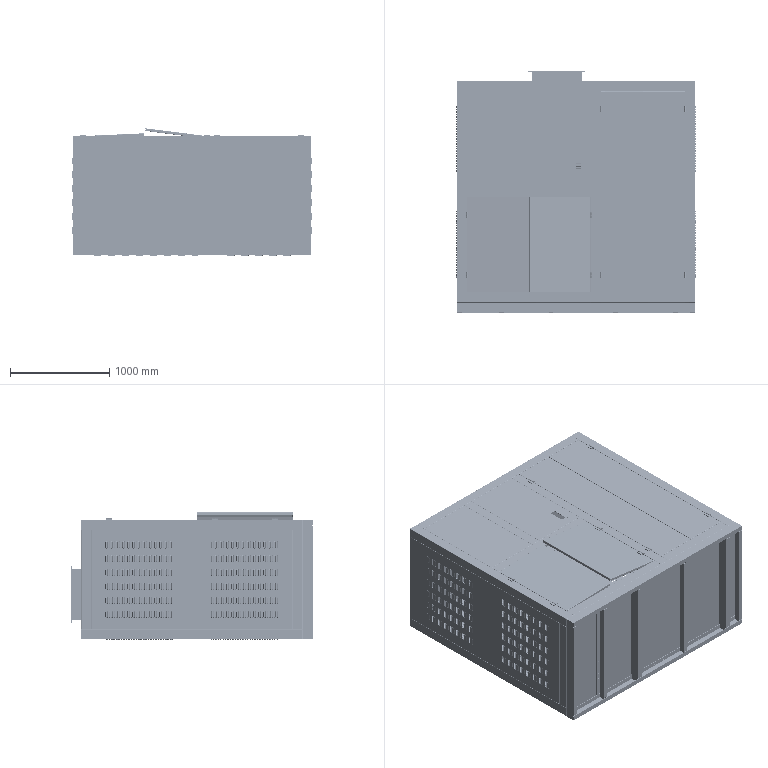Assembly | SolidWorks | mm | 72 component files | 72 solids | 24207 faces | box 2410 x 2430 x 1283.11 mm | volume 69516636 mm3 | plane 10005 | torus 8000 | cylinder 5962 | spline 224 | sphere 16 | commonest cylinder face diameters 10 x3164 14 x2000 2 x288 6 x240 8 x132 12 x64 16 x64 7.5 x4
Bill of materials:
01FrontBase | 1 |  | Long, straight, thin-walled U-channel shown with the open side facing down. It has a flat web and two short side flanges, and no visible holes.
02RearBase | 1 |  | Long, straight, thin-walled U-channel shown with the open side facing up. Small holes are spaced along the flanges, near their top edges.
03LeftSideBase | 1 |  | Straight C-channel standing vertically, opening to the right. The web and flanges appear to end at staggered (offset) heights. One flange has a row of about five small holes.
04RightSideBase | 1 |  | Straight vertical C-channel opening to the left, which appears to be a mirror of the right-opening channels. It has staggered end edges and no visible holes.
05TransformerBaseI | 1 |  | Straight vertical C-channel opening to the right, similar to unnamed part. Its flange holes are in a different pattern: one near the top and three grouped lower down.
06TransformerBaseII | 1 |  | Straight vertical C-channel opening to the left, with staggered ends and no visible holes. It looks the same as unnamed part.
07ResistorBaseI | 1 |  | Straight vertical C-channel opening to the right, similar to the other right-opening channels. It has about four small holes along one flange, spaced fairly evenly in pairs.
08ResistorBaseII | 1 |  | Straight vertical C-channel opening to the left, with staggered ends and no visible holes. It looks the same as unnamed part and unnamed part.
09LeftFrontColumn | 1 |  | Long, straight profile with a stepped, folded cross-section. The end view shows an L-shaped plate with three large round holes, plus thin bent-flange outlines in a Z-like form. Many small holes run along the length, and there are holes near the ends.
10RightFrontColumn | 1 |  | Long, straight profile that appears to be a mirror of unnamed part. The end view shows an L-shaped face with three large holes and Z-like flange outlines. It has fewer holes along its length, mainly small pairs near each end, plus holes on the end face.
11LeftRearColumn | 1 |  | Long, open channel-like profile with stepped or offset flanges. At both ends it has short tabs with small holes, and small holes on the end faces. The end view shows an L-shaped face with three large holes.
12RightRearColumn | 1 |  | Long profile similar to unnamed part, apparently mirrored. It has a row of small holes along one flange, a notched or cut-back flange near the ends, and an end face with holes. The end view shows an L-shaped face with three large holes.
13FrontUpperBeam | 1 |  | Long, straight, thin-walled profile with a right-angle (corner) cross-section. Each leg ends in an outward stepped (Z-jog) flange. An L-shaped end plate with a mitred corner and three round holes closes the end.
14RearUpperBeam | 1 |  | Long, straight, thin-walled right-angle profile with joggled outward flanges on both legs. An L-shaped end plate with three round holes closes the end. It looks like a mirrored or rotated version of the similar long corner profile.
15UpperLeftBeam | 1 |  | Vertical, thin-walled post with a right-angle corner cross-section and joggled outward flanges. L-shaped end plates with three holes sit at the top and bottom.
16UpperRightBeam | 1 |  | Vertical, thin-walled corner-section post with joggled outward flanges and L-shaped end plates with three holes. It appears to be a mirror or rotation of the other corner post.
17FrontMiddleColumn | 1 |  | Long, straight hat-section (top-hat) profile: a raised rectangular channel with an outward flange on each side. A closed end face has two round holes.
18RearMiddleColumn | 1 |  | Long, straight hat-section profile shown inverted, with the channel opening upward and outward flanges at the top. A closed end face has two round holes.
19MiddleUpperBeam | 1 |  | Vertical hat-section post with outward flanges on both sides. End faces at the top and bottom each have two round holes.
20LeftMiddleBeam | 2 |  | Vertical hat-section post: a central channel with an offset flange on each side. End faces at the top and bottom each have two holes.
22BaseLeftSidePlate | 1 |  | Vertical, thin-walled member with a rectangular channel body and a single joggled flange on one side (Z-like, one-sided step). The end face has two round holes.
23BaseRightSidePlate | 1 |  | Vertical, thin-walled member with a channel body and one offset flange on the opposite side from the similar part (mirrored Z-like section). The end face has two round holes.
24BaseFrontSidePlateI | 1 |  | Long, straight, thin-walled profile with a rectangular channel body and one stepped (Z-jog) flange along one edge. The end face has two round holes.
25BaseFrontSidePlateII | 1 |  | Straight, thin-walled profile with a rectangular channel body and one stepped flange along one edge. The end face has two round holes. It appears relatively shorter or wider than the similar long profile.
26BaseRearSidePlateI | 1 |  | Long, slender sheet-metal-style channel with a U-shaped cross-section. One side wall ends in an outward-turned horizontal flange, so the profile looks like a stepped or J shape. The ends are closed by end walls that have holes in them.
27BaseRearSidePlateII | 1 |  | Long sheet-metal-style channel with a U-shaped cross-section, one outward horizontal flange along one side wall, and closed end walls with holes. Similar to part-1f641060 but with fewer side holes.
28FrontMiddleBeam | 1 |  | Long hat-section (omega-profile) channel: a raised crown with two vertical walls and an outward horizontal flange at the base of each wall. The ends are closed by end plates with two holes each.
29RearMiddleBeam | 1 |  | Long hat-section channel shown upside down compared with the previous part: a U-shaped trough with outward horizontal flanges at the top edges. Both ends have end walls with two holes each.
30RearMiddleBeamII | 1 |  | Hat-section trough with outward top flanges and end walls at both ends. It is like part-0d367abd but its side walls have holes, and it looks relatively wider in the top view.
31FrontMiddleColumn | 1 |  | Hat-section channel with the crown on top and outward base flanges. The end walls have two holes each, and there are three small holes along each side wall.
32FrontDoorUpperLeftPlate | 1 |  | Flat rectangular panel or shallow tray with short folded edges around the outside. The edge faces have small, evenly spaced holes. The top face is plain.
33FrontDoorUpperRightPlate | 1 |  | Rectangular panel or shallow tray with short edges and small holes in the edge faces, like part-73c243e1. It also has a rectangular cut-out with four small holes around it near one corner of the top face.
34LeftFront | 1 |  | Rectangular panel with a shallow rim. Along one long edge, a stepped (Z-shaped) offset flange sticks out beyond the main outline. There are two pairs of small holes near the opposite long edge.
35RightFrontDoor | 1 |  | Rectangular panel with a thin perimeter rim and no offset flange. There are two pairs of small holes near one long edge, close to its ends.
36ResistorLeftFrontDoor | 1 |  | Long, narrow rectangular panel with a stepped (Z-shaped) offset flange along one long edge. There are two pairs of small holes near the ends of the other long edge.
37ResistorRightFrontDoor | 1 |  | Long, narrow, flat rectangular panel with a thin edge rim and no offset flange. There are two pairs of small holes near one long edge, at the ends.
38SidePlate | 4 |  | Rectangular thin panel with a shallow perimeter return flange and six parallel rows of closely spaced louver-style slots across the face.
39RearCoverI | 2 |  | Near-square shallow tray-like panel with a perimeter flange and five parallel bands of louver-style slots.
40RearCoverII | 2 |  | Rectangular shallow tray-like panel with a perimeter flange and eight parallel bands of louver-style slots.
41TopPlateI | 1 |  | Plain rectangular panel with a shallow perimeter flange and a ring of small holes near the edges; no other openings.
42TopPlateII | 1 |  | Rectangular panel with a shallow perimeter flange, small perimeter holes, and one large square/rectangular through-cutout offset toward one corner.
43BottomPlate | 1 |  | Very thin flat rectangular sheet with no flanges, perforated by small holes arranged in four vertical column groups.
ActuatorGasket | 1 |  | Elongated rectangular cover with bent-down flanges on the edges, a rectangular through-cutout near one end surrounded by four small holes, and one larger round hole in an end flange.
ColumnBlockingPlate | 4 |  | Bent sheet bracket: a large flat plate with a short perpendicular base tab and a perpendicular side tab, each tab carrying one round hole.
DoorHinge1 | 8 |  | Small rectangular block/plate with rounded edges, two hollow cylindrical knuckles along one long edge, and two cylindrical pins projecting from the underside.
DoorHinge2 | 8 |  | Rectangular block/plate with two hollow cylindrical knuckles offset along one long edge and two cylindrical pins on the underside; similar to, but laid out differently from, unnamed part.
DoorHinge3 | 2 |  | Plain solid cylindrical rod with flat ends and no visible features.
Riser | 1 |  | Open rectangular sleeve/frame (four walls, open both ends) with a thin outward perimeter flange at one end.
Mates:
1. coincident | 03LeftSideBase-2 face at (-123.527, -39.54, 1231.607) dir (0, 1, 0) | 01FrontBase-1 face at (2276.473, -39.54, 1237.107) dir (0, 1, 0)
2. coincident | 03LeftSideBase-2 face at (-75.527, -45.04, 1231.607) dir (0, 0, 1) | 01FrontBase-1 face at (2276.473, -139.54, 1231.607) dir (0, 0, -1)
3. coincident | 03LeftSideBase-2 face at (-123.527, -139.54, 1231.607) dir (-1, 0, 0) | 01FrontBase-1 face at (-123.527, -45.04, 1189.107) dir (-1, 0, 0)
4. coincident | 03LeftSideBase-2 face at (-75.527, -45.04, 42.607) dir (0, 0, -1) | 02RearBase-1 face at (-123.527, -139.54, 42.607) dir (0, 0, 1)
5. coincident | 03LeftSideBase-2 face at (-123.527, -39.54, 1231.607) dir (0, 1, 0) | 02RearBase-1 face at (-123.527, -39.54, 37.107) dir (0, 1, 0)
6. coincident | 03LeftSideBase-2 face at (-123.527, -139.54, 1231.607) dir (-1, 0, 0) | 02RearBase-1 face at (-123.527, -45.04, 85.107) dir (-1, 0, 0)
7. coincident | 01FrontBase-1 face at (2276.473, -45.04, 1189.107) dir (1, 0, 0) | 04RightSideBase-3 face at (2276.473, -139.54, 42.607) dir (1, 0, 0)
8. coincident | 01FrontBase-1 face at (2276.473, -39.54, 1237.107) dir (0, 1, 0) | 04RightSideBase-3 face at (2276.473, -39.54, 42.607) dir (0, 1, 0)
9. coincident | 02RearBase-1 face at (-123.527, -139.54, 42.607) dir (0, 0, 1) | 04RightSideBase-3 face at (2228.473, -45.04, 42.607) dir (0, 0, -1)
10. coincident | 02RearBase-1 face at (-123.527, -39.54, 37.107) dir (0, 1, 0) | 05TransformerBaseI-1 face at (801.473, -39.54, 1231.607) dir (0, 1, 0)
11. coincident | 02RearBase-1 face at (-123.527, -139.54, 42.607) dir (0, 0, 1) | 05TransformerBaseI-1 face at (849.473, -45.04, 42.607) dir (0, 0, -1)
12. coincident | 02RearBase-1 face at (-123.527, -39.54, 37.107) dir (0, 1, 0) | 06TransformerBaseII-1 face at (351.473, -39.54, 42.607) dir (0, 1, 0)
13. coincident | 01FrontBase-1 face at (2276.473, -139.54, 1231.607) dir (0, 0, -1) | 06TransformerBaseII-1 face at (303.473, -45.04, 1231.607) dir (0, 0, 1)
14. coincident | 02RearBase-1 face at (-123.527, -39.54, 37.107) dir (0, 1, 0) | 07ResistorBaseI-1 face at (2053.973, -39.54, 1231.607) dir (0, 1, 0)
15. coincident | 01FrontBase-1 face at (2276.473, -139.54, 1231.607) dir (0, 0, -1) | 07ResistorBaseI-1 face at (2101.973, -45.04, 1231.607) dir (0, 0, 1)
16. coincident | 01FrontBase-1 face at (2276.473, -39.54, 1237.107) dir (0, 1, 0) | 09LeftFrontColumn-2 face at (-95.527, -39.54, 1140.107) dir (0, -1, 0)
17. coincident | 01FrontBase-1 face at (2276.473, -139.54, 1237.107) dir (0, 0, 1) | 09LeftFrontColumn-2 face at (-25.527, 2190.46, 1237.107) dir (0, 0, 1)
18. coincident | 03LeftSideBase-2 face at (-123.527, -139.54, 1231.607) dir (-1, 0, 0) | 09LeftFrontColumn-2 face at (-123.527, 2190.46, 1235.107) dir (-1, 0, 0)
19. coincident | 09LeftFrontColumn-2 face at (-123.527, 2190.46, 1235.107) dir (0, 1, 0) | ColumnBlockingPlate-1 face at (-23.527, 2190.46, 1235.107) dir (0, 1, 0)
20. coincident | 09LeftFrontColumn-2 face at (-121.527, 2190.46, 1235.107) dir (1, 0, 0) | ColumnBlockingPlate-1 face at (-121.527, 2188.46, 1137.107) dir (-1, 0, 0)
21. coincident | 09LeftFrontColumn-2 face at (-25.527, 2190.46, 1235.107) dir (0, 0, -1) | ColumnBlockingPlate-1 face at (-23.527, 2188.46, 1235.107) dir (0, 0, 1)
22. coincident | 04RightSideBase-3 face at (2276.473, -139.54, 42.607) dir (1, 0, 0) | 10RightFrontColumn-1 face at (2276.473, 2190.46, 1139.107) dir (1, 0, 0)
23. coincident | 01FrontBase-1 face at (2276.473, -139.54, 1237.107) dir (0, 0, 1) | 10RightFrontColumn-1 face at (2274.473, 2190.46, 1237.107) dir (0, 0, 1)
24. coincident | 01FrontBase-1 face at (2276.473, -39.54, 1237.107) dir (0, 1, 0) | 10RightFrontColumn-1 face at (2179.473, -39.54, 1209.107) dir (0, -1, 0)
25. coincident | 10RightFrontColumn-1 face at (2274.473, 2190.46, 1235.107) dir (0, 0, -1) | ColumnBlockingPlate-2 face at (2176.473, 2188.46, 1235.107) dir (0, 0, 1)
26. coincident | 10RightFrontColumn-1 face at (2274.473, 2190.46, 1139.107) dir (-1, 0, 0) | ColumnBlockingPlate-2 face at (2274.473, 2188.46, 1137.107) dir (1, 0, 0)
27. coincident | 10RightFrontColumn-1 face at (2273.473, 2190.46, 1234.107) dir (0, 1, 0) | ColumnBlockingPlate-2 face at (2274.473, 2190.46, 1137.107) dir (0, 1, 0)
28. coincident | 03LeftSideBase-2 face at (-123.527, -139.54, 1231.607) dir (-1, 0, 0) | 11LeftRearColumn-1 face at (-123.527, 2190.46, 135.107) dir (-1, 0, 0)
29. coincident | 02RearBase-1 face at (-123.527, -139.54, 37.107) dir (0, 0, -1) | 11LeftRearColumn-1 face at (-121.527, 2190.46, 37.107) dir (0, 0, -1)
30. coincident | 03LeftSideBase-2 face at (-123.527, -39.54, 1231.607) dir (0, 1, 0) | 11LeftRearColumn-1 face at (-26.527, -39.54, 65.107) dir (0, -1, 0)
31. coincident | 11LeftRearColumn-1 face at (-23.527, 2190.46, 39.107) dir (0, 1, 0) | ColumnBlockingPlate-3 face at (-121.527, 2190.46, 137.107) dir (0, 1, 0)
32. coincident | 11LeftRearColumn-1 face at (-121.527, 2190.46, 135.107) dir (1, 0, 0) | ColumnBlockingPlate-3 face at (-121.527, 2188.46, 137.107) dir (-1, 0, 0)
33. coincident | 11LeftRearColumn-1 face at (-121.527, 2190.46, 39.107) dir (0, 0, 1) | ColumnBlockingPlate-3 face at (-23.527, 2188.46, 39.107) dir (0, 0, -1)
34. coincident | 04RightSideBase-3 face at (2276.473, -139.54, 42.607) dir (1, 0, 0) | 12RightRearColumn-2 face at (2276.473, 2190.46, 39.107) dir (1, 0, 0)
35. coincident | 02RearBase-1 face at (-123.527, -139.54, 37.107) dir (0, 0, -1) | 12RightRearColumn-2 face at (2178.473, 2190.46, 37.107) dir (0, 0, -1)
36. coincident | 04RightSideBase-3 face at (2276.473, -39.54, 42.607) dir (0, 1, 0) | 12RightRearColumn-2 face at (2248.473, -39.54, 134.107) dir (0, -1, 0)
37. coincident | 12RightRearColumn-2 face at (2276.473, 2190.46, 39.107) dir (0, 1, 0) | ColumnBlockingPlate-4 face at (2176.473, 2190.46, 39.107) dir (0, 1, 0)
38. coincident | 12RightRearColumn-2 face at (2178.473, 2190.46, 39.107) dir (0, 0, 1) | ColumnBlockingPlate-4 face at (2176.473, 2188.46, 39.107) dir (0, 0, -1)
39. coincident | 12RightRearColumn-2 face at (2274.473, 2190.46, 39.107) dir (-1, 0, 0) | ColumnBlockingPlate-4 face at (2274.473, 2188.46, 137.107) dir (1, 0, 0)
40. coincident | 09LeftFrontColumn-2 face at (-25.527, 2190.46, 1237.107) dir (0, 0, 1) | 13FrontUpperBeam-1 face at (2176.473, 2092.46, 1237.107) dir (0, 0, 1)
41. coincident | ColumnBlockingPlate-1 face at (-23.527, 2190.46, 1235.107) dir (0, 1, 0) | 13FrontUpperBeam-1 face at (2176.473, 2190.46, 1235.107) dir (0, 1, 0)
42. coincident | 10RightFrontColumn-1 face at (2176.473, 2190.46, 1235.107) dir (-1, 0, 0) | 13FrontUpperBeam-1 face at (2176.473, 2187.46, 1209.107) dir (1, 0, 0)
43. coincident | ColumnBlockingPlate-4 face at (2176.473, 2190.46, 39.107) dir (0, 1, 0) | 14RearUpperBeam-1 face at (2176.473, 2190.46, 135.107) dir (0, 1, 0)
44. coincident | 12RightRearColumn-2 face at (2178.473, 2190.46, 37.107) dir (0, 0, -1) | 14RearUpperBeam-1 face at (2176.473, 2188.46, 37.107) dir (0, 0, -1)
45. coincident | 12RightRearColumn-2 face at (2176.473, -39.54, 67.107) dir (-1, 0, 0) | 14RearUpperBeam-1 face at (2176.473, 2093.46, 65.107) dir (1, 0, 0)
46. coincident | ColumnBlockingPlate-1 face at (-23.527, 2190.46, 1235.107) dir (0, 1, 0) | 15UpperLeftBeam-1 face at (-25.527, 2190.46, 137.107) dir (0, 1, 0)
47. coincident | 09LeftFrontColumn-2 face at (-121.527, 2190.46, 1137.107) dir (0, 0, -1) | 15UpperLeftBeam-1 face at (-95.527, 2093.46, 1137.107) dir (0, 0, 1)
48. coincident | 11LeftRearColumn-1 face at (-93.527, -39.54, 137.107) dir (0, 0, 1) | 15UpperLeftBeam-1 face at (-95.527, 2093.46, 137.107) dir (0, 0, -1)
49. coincident | 11LeftRearColumn-1 face at (-123.527, 2190.46, 135.107) dir (-1, 0, 0) | 15UpperLeftBeam-1 face at (-123.527, 2188.46, 137.107) dir (-1, 0, 0)
50. coincident | 02RearBase-1 face at (-123.527, -39.54, 37.107) dir (0, 1, 0) | 18RearMiddleColumn-2 face at (1323.473, -39.54, 39.107) dir (0, -1, 0)
51. coincident | 02RearBase-1 face at (-123.527, -139.54, 37.107) dir (0, 0, -1) | 18RearMiddleColumn-2 face at (1324.473, -39.54, 37.107) dir (0, 0, -1)
52. distance | 18RearMiddleColumn-2 face at (1326.473, 2090.46, 67.107) dir (1, 0, 0) | 12RightRearColumn-2 face at (2276.473, 2190.46, 39.107) dir (1, 0, 0)
53. coincident | 01FrontBase-1 face at (2276.473, -39.54, 1237.107) dir (0, 1, 0) | 17FrontMiddleColumn-2 face at (1229.473, -39.54, 1235.107) dir (0, -1, 0)
54. coincident | 01FrontBase-1 face at (2276.473, -139.54, 1237.107) dir (0, 0, 1) | 17FrontMiddleColumn-2 face at (1228.473, -39.54, 1237.107) dir (0, 0, 1)
55. distance | 17FrontMiddleColumn-2 face at (1326.473, -39.54, 1235.107) dir (1, 0, 0) | 10RightFrontColumn-1 face at (2276.473, 2190.46, 1139.107) dir (1, 0, 0)
56. coincident | 14RearUpperBeam-1 face at (2176.473, 2190.46, 135.107) dir (0, 1, 0) | 16UpperRightBeam-1 face at (2178.473, 2190.46, 1137.107) dir (0, 1, 0)
57. coincident | 12RightRearColumn-2 face at (2276.473, 2190.46, 39.107) dir (1, 0, 0) | 16UpperRightBeam-1 face at (2276.473, 2188.46, 1137.107) dir (1, 0, 0)
58. coincident | 12RightRearColumn-2 face at (2274.473, 2190.46, 137.107) dir (0, 0, 1) | 16UpperRightBeam-1 face at (2248.473, 2093.46, 137.107) dir (0, 0, -1)
59. coincident | 14RearUpperBeam-1 face at (-23.527, 2160.46, 137.107) dir (0, 0, 1) | 19MiddleUpperBeam-1 face at (1323.473, 2188.46, 137.107) dir (0, 0, -1)
60. coincident | 13FrontUpperBeam-1 face at (2176.473, 2190.46, 1235.107) dir (0, 1, 0) | 19MiddleUpperBeam-1 face at (1228.473, 2190.46, 1137.107) dir (0, 1, 0)
61. distance | 19MiddleUpperBeam-1 face at (1226.473, 2160.46, 137.107) dir (-1, 0, 0) | 15UpperLeftBeam-1 face at (-23.527, 2160.46, 1137.107) dir (1, 0, 0)
62. coincident | 11LeftRearColumn-1 face at (-93.527, -39.54, 137.107) dir (0, 0, 1) | 20LeftMiddleBeam-1 face at (-121.527, 1122.46, 137.107) dir (0, 0, -1)
63. coincident | 11LeftRearColumn-1 face at (-123.527, 2190.46, 135.107) dir (-1, 0, 0) | 20LeftMiddleBeam-1 face at (-123.527, 1027.46, 1137.107) dir (-1, 0, 0)
64. distance | 03LeftSideBase-2 face at (-123.527, -39.54, 1231.607) dir (0, 1, 0) | 20LeftMiddleBeam-1 face at (-93.527, 1025.46, 137.107) dir (0, -1, 0)
65. coincident | 12RightRearColumn-2 face at (2276.473, 2190.46, 39.107) dir (1, 0, 0) | 20LeftMiddleBeam-2 face at (2276.473, 1027.46, 137.107) dir (1, 0, 0)
66. coincident | 10RightFrontColumn-1 face at (2246.473, -39.54, 1137.107) dir (0, 0, -1) | 20LeftMiddleBeam-2 face at (2274.473, 1122.46, 1137.107) dir (0, 0, 1)
67. distance | 04RightSideBase-3 face at (2276.473, -39.54, 42.607) dir (0, 1, 0) | 20LeftMiddleBeam-2 face at (2246.473, 1025.46, 1137.107) dir (0, -1, 0)
68. coincident | 09LeftFrontColumn-2 face at (-121.527, 2190.46, 1137.107) dir (0, 0, -1) | 22BaseLeftSidePlate-1 face at (-91.527, -5039.54, 1137.107) dir (0, 0, 1)
69. coincident | 03LeftSideBase-2 face at (-123.527, -39.54, 1231.607) dir (0, 1, 0) | 22BaseLeftSidePlate-1 face at (-91.527, -39.54, -4862.893) dir (0, -1, 0)
70. coincident | 03LeftSideBase-2 face at (-123.527, -139.54, 1231.607) dir (-1, 0, 0) | 22BaseLeftSidePlate-1 face at (-123.527, 60.46, 1137.107) dir (-1, 0, 0)
71. coincident | 04RightSideBase-3 face at (2276.473, -139.54, 42.607) dir (1, 0, 0) | 23BaseRightSidePlate-1 face at (2276.473, 60.46, 137.107) dir (1, 0, 0)
72. coincident | 04RightSideBase-3 face at (2276.473, -39.54, 42.607) dir (0, 1, 0) | 23BaseRightSidePlate-1 face at (2244.473, -39.54, 6137.107) dir (0, -1, 0)
73. coincident | 10RightFrontColumn-1 face at (2246.473, -39.54, 1137.107) dir (0, 0, -1) | 23BaseRightSidePlate-1 face at (2244.473, 5060.46, 1137.107) dir (0, 0, 1)
74. coincident | 01FrontBase-1 face at (2276.473, -139.54, 1237.107) dir (0, 0, 1) | 24BaseFrontSidePlateI-1 face at (1226.473, 60.46, 1237.107) dir (0, 0, 1)
75. coincident | 17FrontMiddleColumn-2 face at (1226.473, 2090.46, 1207.107) dir (-1, 0, 0) | 24BaseFrontSidePlateI-1 face at (1226.473, -6289.54, 1205.107) dir (1, 0, 0)
76. coincident | 01FrontBase-1 face at (2276.473, -39.54, 1237.107) dir (0, 1, 0) | 24BaseFrontSidePlateI-1 face at (-6273.527, -39.54, 1205.107) dir (0, -1, 0)
77. coincident | 10RightFrontColumn-1 face at (2176.473, 2190.46, 1235.107) dir (-1, 0, 0) | 25BaseFrontSidePlateII-1 face at (2176.473, -4289.54, 1205.107) dir (1, 0, 0)
78. coincident | 01FrontBase-1 face at (2276.473, -139.54, 1237.107) dir (0, 0, 1) | 25BaseFrontSidePlateII-1 face at (2176.473, 60.46, 1237.107) dir (0, 0, 1)
79. coincident | 01FrontBase-1 face at (2276.473, -39.54, 1237.107) dir (0, 1, 0) | 25BaseFrontSidePlateII-1 face at (-2923.527, -39.54, 1205.107) dir (0, -1, 0)
80. coincident | 18RearMiddleColumn-2 face at (1226.473, -39.54, 39.107) dir (-1, 0, 0) | 26BaseRearSidePlateI-1 face at (1226.473, 6310.46, 69.107) dir (1, 0, 0)
81. coincident | 02RearBase-1 face at (-123.527, -139.54, 37.107) dir (0, 0, -1) | 26BaseRearSidePlateI-1 face at (-23.527, 60.46, 37.107) dir (0, 0, -1)
82. coincident | 02RearBase-1 face at (-123.527, -39.54, 37.107) dir (0, 1, 0) | 26BaseRearSidePlateI-1 face at (7476.473, -39.54, 69.107) dir (0, -1, 0)
83. coincident | 02RearBase-1 face at (-123.527, -139.54, 37.107) dir (0, 0, -1) | 27BaseRearSidePlateII-1 face at (1326.473, 60.46, 37.107) dir (0, 0, -1)
84. coincident | 18RearMiddleColumn-2 face at (1326.473, 2090.46, 67.107) dir (1, 0, 0) | 27BaseRearSidePlateII-1 face at (1326.473, -4289.54, 69.107) dir (-1, 0, 0)
85. coincident | 02RearBase-1 face at (-123.527, -39.54, 37.107) dir (0, 1, 0) | 27BaseRearSidePlateII-1 face at (6426.473, -39.54, 69.107) dir (0, -1, 0)
86. coincident | 09LeftFrontColumn-2 face at (-25.527, 2190.46, 1237.107) dir (0, 0, 1) | 28FrontMiddleBeam-1 face at (1226.473, 1027.46, 1237.107) dir (0, 0, 1)
87. coincident | 09LeftFrontColumn-2 face at (-23.527, -39.54, 1207.107) dir (1, 0, 0) | 28FrontMiddleBeam-1 face at (-23.527, 1122.46, 1235.107) dir (-1, 0, 0)
88. distance | 28FrontMiddleBeam-1 face at (-23.527, 1025.46, 1207.107) dir (0, -1, 0) | 24BaseFrontSidePlateI-1 face at (7476.473, 60.46, 1205.107) dir (0, 1, 0)
89. coincident | 11LeftRearColumn-1 face at (-23.527, 2190.46, 39.107) dir (1, 0, 0) | 29RearMiddleBeam-1 face at (-23.527, 1028.46, 39.107) dir (-1, 0, 0)
90. distance | 26BaseRearSidePlateI-1 face at (-6273.527, 60.46, 69.107) dir (0, 1, 0) | 29RearMiddleBeam-1 face at (1226.473, 1025.46, 67.107) dir (0, -1, 0)
91. coincident | 12RightRearColumn-2 face at (2176.473, -39.54, 67.107) dir (-1, 0, 0) | 30RearMiddleBeamII-1 face at (2176.473, 1122.46, 39.107) dir (1, 0, 0)
92. distance | 27BaseRearSidePlateII-1 face at (-2923.527, 60.46, 69.107) dir (0, 1, 0) | 30RearMiddleBeamII-1 face at (2176.473, 1025.46, 39.107) dir (0, -1, 0)
93. coincident | 28FrontMiddleBeam-1 face at (1226.473, 1027.46, 1237.107) dir (0, 0, 1) | 31FrontMiddleColumn-1 face at (553.473, 1125.46, 1237.107) dir (0, 0, 1)
94. coincident | 28FrontMiddleBeam-1 face at (1226.473, 1125.46, 1235.107) dir (0, 1, 0) | 31FrontMiddleColumn-1 face at (554.473, 1125.46, 1235.107) dir (0, -1, 0)
95. distance | 31FrontMiddleColumn-1 face at (651.473, 1125.46, 1235.107) dir (1, 0, 0) | 17FrontMiddleColumn-2 face at (1226.473, 2090.46, 1207.107) dir (-1, 0, 0)
96. coincident | 28FrontMiddleBeam-1 face at (1226.473, 1125.46, 1235.107) dir (0, 1, 0) | 33FrontDoorUpperRightPlate-1 face at (-4173.527, 1125.46, 1209.107) dir (0, -1, 0)
97. coincident | 31FrontMiddleColumn-1 face at (651.473, 1125.46, 1235.107) dir (1, 0, 0) | 33FrontDoorUpperRightPlate-1 face at (651.473, 6915.46, 1209.107) dir (-1, 0, 0)
98. coincident | 31FrontMiddleColumn-1 face at (553.473, 1125.46, 1237.107) dir (0, 0, 1) | 33FrontDoorUpperRightPlate-1 face at (651.473, 2090.46, 1237.107) dir (0, 0, 1)
99. coincident | 09LeftFrontColumn-2 face at (-23.527, -39.54, 1207.107) dir (1, 0, 0) | 32FrontDoorUpperLeftPlate-2 face at (-23.527, 6915.46, 1209.107) dir (-1, 0, 0)
100. coincident | 28FrontMiddleBeam-1 face at (1226.473, 1125.46, 1235.107) dir (0, 1, 0) | 32FrontDoorUpperLeftPlate-2 face at (-4848.527, 1125.46, 1209.107) dir (0, -1, 0)
101. coincident | 09LeftFrontColumn-2 face at (-25.527, 2190.46, 1237.107) dir (0, 0, 1) | 32FrontDoorUpperLeftPlate-2 face at (-23.527, 2090.46, 1237.107) dir (0, 0, 1)
102. coincident | 12RightRearColumn-2 face at (2276.473, 2190.46, 39.107) dir (1, 0, 0) | 38SidePlate-1 face at (2276.473, 2090.46, 1137.107) dir (1, 0, 0)
103. coincident | 16UpperRightBeam-1 face at (2274.473, 2090.46, 1137.107) dir (0, -1, 0) | 38SidePlate-1 face at (2248.473, 2090.46, -4862.893) dir (0, 1, 0)
104. coincident | 10RightFrontColumn-1 face at (2246.473, -39.54, 1137.107) dir (0, 0, -1) | 38SidePlate-1 face at (2248.473, 7090.46, 1137.107) dir (0, 0, 1)
105. coincident | 12RightRearColumn-2 face at (2276.473, 2190.46, 39.107) dir (1, 0, 0) | 38SidePlate-2 face at (2276.473, 1025.46, 1137.107) dir (1, 0, 0)
106. coincident | 23BaseRightSidePlate-1 face at (2244.473, 60.46, -4862.893) dir (0, 1, 0) | 38SidePlate-2 face at (2248.473, 60.46, 6137.107) dir (0, -1, 0)
107. coincident | 10RightFrontColumn-1 face at (2246.473, -39.54, 1137.107) dir (0, 0, -1) | 38SidePlate-2 face at (2248.473, 6025.46, 1137.107) dir (0, 0, 1)
108. coincident | 11LeftRearColumn-1 face at (-123.527, 2190.46, 135.107) dir (-1, 0, 0) | 38SidePlate-3 face at (-123.527, 2090.46, 137.107) dir (-1, 0, 0)
109. coincident | 15UpperLeftBeam-1 face at (-121.527, 2090.46, 137.107) dir (0, -1, 0) | 38SidePlate-3 face at (-95.527, 2090.46, 6137.107) dir (0, 1, 0)
110. coincident | 09LeftFrontColumn-2 face at (-121.527, 2190.46, 1137.107) dir (0, 0, -1) | 38SidePlate-3 face at (-95.527, -3874.54, 1137.107) dir (0, 0, 1)
111. coincident | 11LeftRearColumn-1 face at (-123.527, 2190.46, 135.107) dir (-1, 0, 0) | 38SidePlate-4 face at (-123.527, 1025.46, 137.107) dir (-1, 0, 0)
112. coincident | 22BaseLeftSidePlate-1 face at (-91.527, 60.46, 6137.107) dir (0, 1, 0) | 38SidePlate-4 face at (-95.527, 60.46, -4862.893) dir (0, -1, 0)
113. coincident | 09LeftFrontColumn-2 face at (-121.527, 2190.46, 1137.107) dir (0, 0, -1) | 38SidePlate-4 face at (-95.527, -4939.54, 1137.107) dir (0, 0, 1)
114. coincident | 18RearMiddleColumn-2 face at (1326.473, 2090.46, 67.107) dir (1, 0, 0) | 39RearCoverI-1 face at (1326.473, -3699.54, 65.107) dir (-1, 0, 0)
115. coincident | 30RearMiddleBeamII-1 face at (1326.473, 1125.46, 67.107) dir (0, 1, 0) | 39RearCoverI-1 face at (7001.473, 1125.46, 65.107) dir (0, -1, 0)
116. coincident | 18RearMiddleColumn-2 face at (1324.473, -39.54, 37.107) dir (0, 0, -1) | 39RearCoverI-2 face at (2176.473, 1025.46, 37.107) dir (0, 0, -1)
117. coincident | 18RearMiddleColumn-2 face at (1326.473, 2090.46, 67.107) dir (1, 0, 0) | 39RearCoverI-2 face at (1326.473, -4764.54, 65.107) dir (-1, 0, 0)
118. coincident | 27BaseRearSidePlateII-1 face at (-2923.527, 60.46, 69.107) dir (0, 1, 0) | 39RearCoverI-2 face at (7001.473, 60.46, 65.107) dir (0, -1, 0)
119. coincident | 18RearMiddleColumn-2 face at (1226.473, -39.54, 39.107) dir (-1, 0, 0) | 40RearCoverII-1 face at (1226.473, 8340.46, 65.107) dir (1, 0, 0)
120. coincident | 14RearUpperBeam-1 face at (2176.473, 2090.46, 39.107) dir (0, -1, 0) | 40RearCoverII-1 face at (-6273.527, 2090.46, 65.107) dir (0, 1, 0)
121. coincident | 11LeftRearColumn-1 face at (-121.527, 2190.46, 37.107) dir (0, 0, -1) | 40RearCoverII-2 face at (1226.473, 1025.46, 37.107) dir (0, 0, -1)
122. coincident | 29RearMiddleBeam-1 face at (1226.473, 1025.46, 67.107) dir (0, -1, 0) | 40RearCoverII-2 face at (-6273.527, 1025.46, 65.107) dir (0, 1, 0)
123. coincident | 18RearMiddleColumn-2 face at (1226.473, -39.54, 39.107) dir (-1, 0, 0) | 40RearCoverII-2 face at (1226.473, 7275.46, 65.107) dir (1, 0, 0)
124. coincident | 15UpperLeftBeam-1 face at (-25.527, 2190.46, 137.107) dir (0, 1, 0) | 42TopPlateII-1 face at (-23.527, 2190.46, 137.107) dir (0, 1, 0)
125. coincident | 14RearUpperBeam-1 face at (-23.527, 2160.46, 137.107) dir (0, 0, 1) | 42TopPlateII-1 face at (7476.473, 2162.46, 137.107) dir (0, 0, -1)
126. coincident | 15UpperLeftBeam-1 face at (-23.527, 2160.46, 1137.107) dir (1, 0, 0) | 42TopPlateII-1 face at (-23.527, 2162.46, -6112.893) dir (-1, 0, 0)
127. coincident | 16UpperRightBeam-1 face at (2178.473, 2190.46, 1137.107) dir (0, 1, 0) | 41TopPlateI-1 face at (1326.473, 2190.46, 137.107) dir (0, 1, 0)
128. coincident | 16UpperRightBeam-1 face at (2176.473, 2160.46, 137.107) dir (-1, 0, 0) | 41TopPlateI-1 face at (2176.473, 2162.46, 6137.107) dir (1, 0, 0)
129. coincident | 42TopPlateII-1 face at (-23.527, 2190.46, 137.107) dir (0, 1, 0) | Riser-1 face at (1134.473, 2190.46, -18.299) dir (0, -1, 0)
130. distance | 16UpperRightBeam-1 face at (2276.473, 2188.46, 1137.107) dir (1, 0, 0) | Riser-1 face at (1131.473, 2190.46, -18.299) dir (-1, 0, 0)
131. distance | Riser-1 face at (1131.473, 2190.46, 237.107) dir (0, 0, 1) | 14RearUpperBeam-1 face at (2176.473, 2188.46, 37.107) dir (0, 0, -1)
132. coincident | 18RearMiddleColumn-2 face at (1324.473, -39.54, 37.107) dir (0, 0, -1) | 30RearMiddleBeamII-1 face at (2176.473, 1123.46, 37.107) dir (0, 0, -1)
133. coincident | 11LeftRearColumn-1 face at (-121.527, 2190.46, 37.107) dir (0, 0, -1) | 29RearMiddleBeam-1 face at (-23.527, 1027.46, 37.107) dir (0, 0, -1)
134. coincident | 11LeftRearColumn-1 face at (-121.527, 2190.46, 37.107) dir (0, 0, -1) | 40RearCoverII-1 face at (1226.473, 2090.46, 37.107) dir (0, 0, -1)
135. coincident | 12RightRearColumn-2 face at (2178.473, 2190.46, 37.107) dir (0, 0, -1) | 39RearCoverI-1 face at (1326.473, 1125.46, 37.107) dir (0, 0, -1)
136. distance | 06TransformerBaseII-1 face at (351.473, -139.54, 42.607) dir (1, 0, 0) | 03LeftSideBase-2 face at (-123.527, -139.54, 1231.607) dir (-1, 0, 0)
137. distance | 07ResistorBaseI-1 face at (2053.973, -139.54, 1231.607) dir (-1, 0, 0) | 04RightSideBase-3 face at (2276.473, -139.54, 42.607) dir (1, 0, 0)
138. distance | 43BottomPlate-1 face at (-93.527, -36.54, 1207.107) dir (0, 0, 1) | 01FrontBase-1 face at (2276.473, -139.54, 1237.107) dir (0, 0, 1)
139. distance | 43BottomPlate-1 face at (-93.527, -36.54, 67.107) dir (-1, 0, 0) | 03LeftSideBase-2 face at (-123.527, -139.54, 1231.607) dir (-1, 0, 0)
140. coincident | 04RightSideBase-3 face at (2276.473, -39.54, 42.607) dir (0, 1, 0) | 43BottomPlate-1 face at (-93.527, -39.54, 1207.107) dir (0, -1, 0)
141. distance | 07ResistorBaseI-1 face at (2053.973, -139.54, 1231.607) dir (-1, 0, 0) | 08ResistorBaseII-1 face at (1448.973, -39.54, 42.607) dir (-1, 0, 0)
142. coincident | 07ResistorBaseI-1 face at (2053.973, -39.54, 1231.607) dir (0, 1, 0) | 08ResistorBaseII-1 face at (1496.973, -39.54, 42.607) dir (0, 1, 0)
143. coincident | 07ResistorBaseI-1 face at (2101.973, -114.351, 1181.607) dir (0, 0, 1) | 08ResistorBaseII-1 face at (1448.973, -114.351, 1181.607) dir (0, 0, 1)
144. concentric | 10RightFrontColumn-1 edge at (2192.973, 1927.96, 1237.107) dir (0, 0, 1) r 5 | DoorHinge1-1 face at (2192.973, 1927.96, 1224.607) dir (0, 0, 1) r 4
145. concentric | 10RightFrontColumn-1 face at (2192.973, 1892.96, 1112.106) dir (0, 0, 1) r 5 | DoorHinge1-1 face at (2192.973, 1892.96, 1224.607) dir (0, 0, 1) r 4
146. coincident | 10RightFrontColumn-1 face at (2274.473, 2190.46, 1237.107) dir (0, 0, 1) | DoorHinge1-1 face at (2154.261, 1880.46, 1237.107) dir (0, 0, -1)
147. concentric | 37ResistorRightFrontDoor-1 face at (2157.973, 1892.96, 1210.106) dir (0, 0, 1) r 5 | DoorHinge2-1 face at (2157.973, 1892.96, 1224.607) dir (0, 0, 1) r 4
148. concentric | 37ResistorRightFrontDoor-1 face at (2157.973, 1927.96, 1210.106) dir (0, 0, 1) r 5 | DoorHinge2-1 face at (2157.973, 1927.96, 1224.607) dir (0, 0, 1) r 4
149. coincident | 37ResistorRightFrontDoor-1 face at (1753.473, 2088.46, 1237.107) dir (0, 0, 1) | DoorHinge2-1 face at (2196.684, 1940.46, 1237.107) dir (0, 0, -1)
150. concentric | DoorHinge1-1 face at (2175.473, 1938.46, 1245.107) dir (0, -1, 0) r 4 | DoorHinge2-1 face at (2175.473, 1880.46, 1245.107) dir (0, 1, 0) r 4
151. coincident | DoorHinge1-1 face at (2167.473, 1910.46, 1295.107) dir (0, 1, 0) | DoorHinge2-1 face at (2167.473, 1910.46, 1295.107) dir (0, -1, 0)
152. coincident | DoorHinge1-1 face at (2175.473, 1938.46, 1245.107) dir (0, -1, 0) | DoorHinge3-1 face at (2175.473, 1938.46, 1245.107) dir (0, 1, 0)
153. coincident | 37ResistorRightFrontDoor-1 face at (1753.473, 2088.46, 1237.107) dir (0, 0, 1) | DoorHinge2-2 face at (2196.684, 270.46, 1237.107) dir (0, 0, -1)
154. concentric | 37ResistorRightFrontDoor-1 face at (2157.973, 257.96, 1210.106) dir (0, 0, 1) r 5 | DoorHinge2-2 face at (2157.973, 257.96, 1224.607) dir (0, 0, 1) r 4
155. concentric | 37ResistorRightFrontDoor-1 face at (2157.973, 222.96, 1210.106) dir (0, 0, 1) r 5 | DoorHinge2-2 face at (2157.973, 222.96, 1224.607) dir (0, 0, 1) r 4
156. concentric | 10RightFrontColumn-1 edge at (2192.973, 257.96, 1237.107) dir (0, 0, 1) r 5 | DoorHinge1-2 face at (2192.973, 257.96, 1224.607) dir (0, 0, 1) r 4
157. concentric | 10RightFrontColumn-1 edge at (2192.973, 222.96, 1237.107) dir (0, 0, 1) r 5 | DoorHinge1-2 face at (2192.973, 222.96, 1224.607) dir (0, 0, 1) r 4
158. coincident | 10RightFrontColumn-1 face at (2274.473, 2190.46, 1237.107) dir (0, 0, 1) | DoorHinge1-2 face at (2154.261, 210.46, 1237.107) dir (0, 0, -1)
159. concentric | DoorHinge1-2 face at (2175.473, 210.46, 1245.107) dir (0, 1, 0) r 8 | DoorHinge2-2 face at (2175.473, 270.46, 1245.107) dir (0, -1, 0) r 8
160. concentric | DoorHinge1-1 face at (2175.473, 1938.46, 1245.107) dir (0, -1, 0) r 4 | DoorHinge3-1 face at (2175.473, 1938.46, 1245.107) dir (0, -1, 0) r 4
161. concentric | DoorHinge2-2 face at (2175.473, 210.46, 1245.107) dir (0, 1, 0) r 4 | DoorHinge3-3 face at (2175.473, 268.46, 1245.107) dir (0, -1, 0) r 4
162. coincident | DoorHinge1-2 face at (2175.473, 268.46, 1245.107) dir (0, -1, 0) | DoorHinge3-3 face at (2175.473, 268.46, 1245.107) dir (0, 1, 0)
163. concentric | 17FrontMiddleColumn-2 face at (1309.973, 222.96, 1205.106) dir (0, 0, 1) r 5 | DoorHinge1-3 face at (1309.973, 222.96, 1224.607) dir (0, 0, 1) r 4
164. concentric | 17FrontMiddleColumn-2 face at (1309.973, 257.96, 1205.106) dir (0, 0, 1) r 5 | DoorHinge1-3 face at (1309.973, 257.96, 1224.607) dir (0, 0, 1) r 4
165. coincident | 17FrontMiddleColumn-2 face at (1228.473, -39.54, 1237.107) dir (0, 0, 1) | DoorHinge1-3 face at (1348.684, 270.46, 1237.107) dir (0, 0, -1)
166. concentric | 36ResistorLeftFrontDoor-1 edge at (1344.973, 257.96, 1237.107) dir (0, 0, 1) r 5 | DoorHinge2-3 face at (1344.973, 257.96, 1224.607) dir (0, 0, 1) r 4
167. concentric | 36ResistorLeftFrontDoor-1 edge at (1344.973, 222.96, 1237.107) dir (0, 0, 1) r 5 | DoorHinge2-3 face at (1344.973, 222.96, 1224.607) dir (0, 0, 1) r 4
168. coincident | 36ResistorLeftFrontDoor-1 face at (1328.473, 2088.46, 1237.107) dir (0, 0, 1) | DoorHinge2-3 face at (1306.261, 210.46, 1237.107) dir (0, 0, -1)
169. concentric | DoorHinge1-3 face at (1327.473, 270.46, 1245.107) dir (0, -1, 0) r 8 | DoorHinge2-3 face at (1327.473, 270.46, 1245.107) dir (0, -1, 0) r 4
170. coincident | DoorHinge1-3 face at (1348.684, 270.46, 1245.107) dir (0, 1, 0) | DoorHinge2-3 face at (1306.261, 270.46, 1245.107) dir (0, 1, 0)
171. concentric | DoorHinge1-4 face at (1309.973, 1892.96, 1224.607) dir (0, 0, 1) r 4 | 17FrontMiddleColumn-2 edge at (1309.973, 1892.96, 1237.107) dir (0, 0, 1) r 5
172. concentric | 17FrontMiddleColumn-2 edge at (1309.973, 1927.96, 1237.107) dir (0, 0, 1) r 5 | DoorHinge1-4 face at (1309.973, 1927.96, 1224.607) dir (0, 0, 1) r 4
173. coincident | 17FrontMiddleColumn-2 face at (1228.473, -39.54, 1237.107) dir (0, 0, 1) | DoorHinge1-4 face at (1348.684, 1940.46, 1237.107) dir (0, 0, -1)
174. concentric | 36ResistorLeftFrontDoor-1 edge at (1344.973, 1927.96, 1237.107) dir (0, 0, 1) r 5 | DoorHinge2-4 face at (1344.973, 1927.96, 1224.607) dir (0, 0, 1) r 4
175. concentric | 36ResistorLeftFrontDoor-1 edge at (1344.973, 1892.96, 1237.107) dir (0, 0, 1) r 5 | DoorHinge2-4 face at (1344.973, 1892.96, 1224.607) dir (0, 0, 1) r 4
176. coincident | 36ResistorLeftFrontDoor-1 face at (1328.473, 2088.46, 1237.107) dir (0, 0, 1) | DoorHinge2-4 face at (1306.261, 1880.46, 1237.107) dir (0, 0, -1)
177. concentric | 17FrontMiddleColumn-2 edge at (1242.973, 257.96, 1237.107) dir (0, 0, 1) r 5 | DoorHinge1-5 face at (1242.973, 257.96, 1224.607) dir (0, 0, 1) r 4
178. concentric | 17FrontMiddleColumn-2 edge at (1242.973, 222.96, 1237.107) dir (0, 0, 1) r 5 | DoorHinge1-5 face at (1242.973, 222.96, 1224.607) dir (0, 0, 1) r 4
179. coincident | 17FrontMiddleColumn-2 face at (1228.473, -39.54, 1237.107) dir (0, 0, 1) | DoorHinge1-5 face at (1204.261, 210.46, 1237.107) dir (0, 0, -1)
180. concentric | 35RightFrontDoor-1 edge at (1207.104, 222.96, 1239.377) dir (0.1261, 0, 0.992) r 5 | DoorHinge2-5 face at (1205.528, 222.96, 1226.977) dir (0.1261, 0, 0.992) r 4
181. concentric | 35RightFrontDoor-1 edge at (1207.104, 257.96, 1239.377) dir (0.1261, 0, 0.992) r 5 | DoorHinge2-5 face at (1205.528, 257.96, 1226.977) dir (0.1261, 0, 0.992) r 4
182. coincident | 35RightFrontDoor-1 face at (607.426, 1023.46, 1315.576) dir (0.1261, 0, 0.992) | DoorHinge2-5 face at (1245.507, 270.46, 1234.497) dir (-0.1261, 0, -0.992)
183. concentric | 17FrontMiddleColumn-2 edge at (1242.973, 862.96, 1237.107) dir (0, 0, 1) r 5 | DoorHinge1-6 face at (1242.973, 862.96, 1224.607) dir (0, 0, 1) r 4
184. concentric | 17FrontMiddleColumn-2 edge at (1242.973, 827.96, 1237.107) dir (0, 0, 1) r 5 | DoorHinge1-6 face at (1242.973, 827.96, 1224.607) dir (0, 0, 1) r 4
185. coincident | 17FrontMiddleColumn-2 face at (1228.473, -39.54, 1237.107) dir (0, 0, 1) | DoorHinge1-6 face at (1204.261, 815.46, 1237.107) dir (0, 0, -1)
186. concentric | DoorHinge1-4 face at (1327.473, 1940.46, 1245.107) dir (0, -1, 0) r 8 | DoorHinge2-4 face at (1327.473, 1880.46, 1245.107) dir (0, 1, 0) r 8
187. concentric | 35RightFrontDoor-1 edge at (1207.104, 827.96, 1239.377) dir (0.1261, 0, 0.992) r 5 | DoorHinge2-6 face at (1205.528, 827.96, 1226.977) dir (0.1261, 0, 0.992) r 4
188. concentric | 35RightFrontDoor-1 edge at (1207.104, 862.96, 1239.377) dir (0.1261, 0, 0.992) r 5 | DoorHinge2-6 face at (1205.528, 862.96, 1226.977) dir (0.1261, 0, 0.992) r 4
189. coincident | 35RightFrontDoor-1 face at (607.426, 1023.46, 1315.576) dir (0.1261, 0, 0.992) | DoorHinge2-6 face at (1245.507, 875.46, 1234.497) dir (-0.1261, 0, -0.992)
190. concentric | DoorHinge1-6 face at (1225.473, 815.46, 1245.107) dir (0, 1, 0) r 8 | DoorHinge2-6 face at (1225.473, 875.46, 1245.107) dir (0, -1, 0) r 8
191. coincident | DoorHinge1-5 face at (1204.261, 270.46, 1245.107) dir (0, 1, 0) | DoorHinge2-5 face at (1246.515, 270.46, 1242.434) dir (0, 1, 0)
192. concentric | 09LeftFrontColumn-2 edge at (-40.027, 862.96, 1237.107) dir (0, 0, 1) r 5 | DoorHinge1-7 face at (-40.027, 862.96, 1224.607) dir (0, 0, 1) r 4
193. concentric | 09LeftFrontColumn-2 edge at (-40.027, 827.96, 1237.107) dir (0, 0, 1) r 5 | DoorHinge1-7 face at (-40.027, 827.96, 1224.607) dir (0, 0, 1) r 4
194. coincident | 09LeftFrontColumn-2 face at (-25.527, 2190.46, 1237.107) dir (0, 0, 1) | DoorHinge1-7 face at (-1.316, 875.46, 1237.107) dir (0, 0, -1)
195. concentric | 34LeftFront-2 edge at (-4.677, 862.96, 1237.922) dir (-0.04606, 0, 0.9989) r 5 | DoorHinge2-7 face at (-4.102, 862.96, 1225.435) dir (-0.04606, 0, 0.9989) r 4
196. concentric | 34LeftFront-2 edge at (-4.677, 827.96, 1237.922) dir (-0.04606, 0, 0.9989) r 5 | DoorHinge2-7 face at (-4.102, 827.96, 1225.435) dir (-0.04606, 0, 0.9989) r 4
197. coincident | 34LeftFront-2 face at (-21.16, 1023.46, 1237.162) dir (-0.04606, 0, 0.9989) | DoorHinge2-7 face at (-43.348, 815.46, 1236.139) dir (0.04606, 0, -0.9989)
198. concentric | DoorHinge1-7 edge at (-22.527, 845.46, 1245.107) dir (0, 1, 0) r 4 | DoorHinge2-7 edge at (-22.527, 830.46, 1245.107) dir (0, -1, 0) r 4
199. coincident | DoorHinge1-7 face at (-1.316, 875.46, 1245.107) dir (0, 1, 0) | DoorHinge2-7 face at (-43.716, 875.46, 1244.13) dir (0, 1, 0)
200. concentric | 09LeftFrontColumn-2 edge at (-40.027, 222.96, 1235.107) dir (0, 0, -1) r 4.675 | DoorHinge1-8 face at (-40.027, 222.96, 1224.607) dir (0, 0, 1) r 4
201. concentric | 09LeftFrontColumn-2 edge at (-40.027, 257.96, 1237.107) dir (0, 0, 1) r 5.477 | DoorHinge1-8 face at (-40.027, 257.96, 1224.607) dir (0, 0, 1) r 4
202. coincident | 09LeftFrontColumn-2 face at (-25.527, 2190.46, 1237.107) dir (0, 0, 1) | DoorHinge1-8 face at (-1.316, 270.46, 1237.107) dir (0, 0, -1)
203. concentric | 34LeftFront-2 edge at (-4.677, 257.96, 1237.922) dir (-0.04606, 0, 0.9989) r 5 | DoorHinge2-8 face at (-4.102, 257.96, 1225.435) dir (-0.04606, 0, 0.9989) r 4
204. concentric | 34LeftFront-2 edge at (-4.677, 222.96, 1237.922) dir (-0.04606, 0, 0.9989) r 5 | DoorHinge2-8 face at (-4.102, 222.96, 1225.435) dir (-0.04606, 0, 0.9989) r 4
205. coincident | 34LeftFront-2 face at (-21.16, 1023.46, 1237.162) dir (-0.04606, 0, 0.9989) | DoorHinge2-8 face at (-43.348, 210.46, 1236.139) dir (0.04606, 0, -0.9989)
206. coincident | 14RearUpperBeam-1 face at (-23.527, 2160.46, 137.107) dir (0, 0, 1) | 41TopPlateI-1 face at (7176.473, 2162.46, 137.107) dir (0, 0, -1)
207. coincident | 13FrontUpperBeam-1 face at (2176.473, 2092.46, 1237.107) dir (0, 0, 1) | 36ResistorLeftFrontDoor-1 face at (1328.473, 2088.46, 1237.107) dir (0, 0, 1)
208. coincident | 13FrontUpperBeam-1 face at (2176.473, 2092.46, 1237.107) dir (0, 0, 1) | 37ResistorRightFrontDoor-1 face at (1753.473, 2088.46, 1237.107) dir (0, 0, 1)
209. coincident | 33FrontDoorUpperRightPlate-1 face at (651.473, 2090.46, 1235.107) dir (0, 0, -1) | ActuatorGasket-1 face at (1223.973, 1425.46, 1235.107) dir (0, 0, 1)
210. distance | ActuatorGasket-1 face at (1125.973, 1221.96, 1235.108) dir (0, 1, 0) | 01FrontBase-1 face at (2276.473, -139.54, 1189.107) dir (0, -1, 0)
211. distance | 33FrontDoorUpperRightPlate-1 face at (1224.473, -3699.54, 1209.107) dir (-1, 0, 0) | ActuatorGasket-1 face at (1223.973, -1674.54, 1211.107) dir (1, 0, 0)
212. distance | 06TransformerBaseII-1 face at (351.473, -139.54, 42.607) dir (1, 0, 0) | 05TransformerBaseI-1 face at (849.473, -39.54, 1231.607) dir (1, 0, 0)